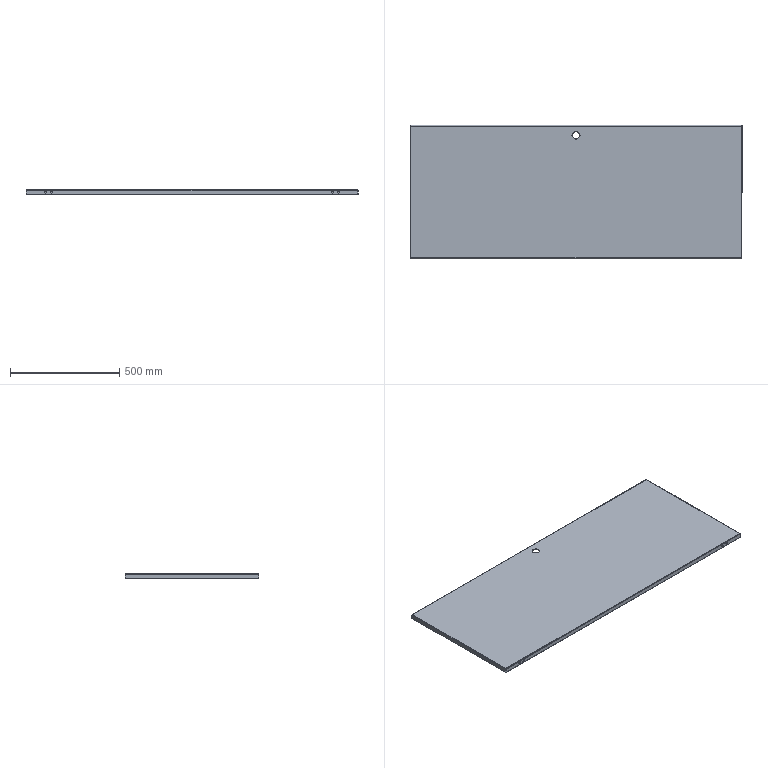Component | SolidWorks | Door-1 | 1 solid | 83 faces | volume 1997572 mm3 | plane 54 | cylinder 29 | commonest cylinder face diameters 5 x9 8.5 x8 32 x4 6 x4 2 x4